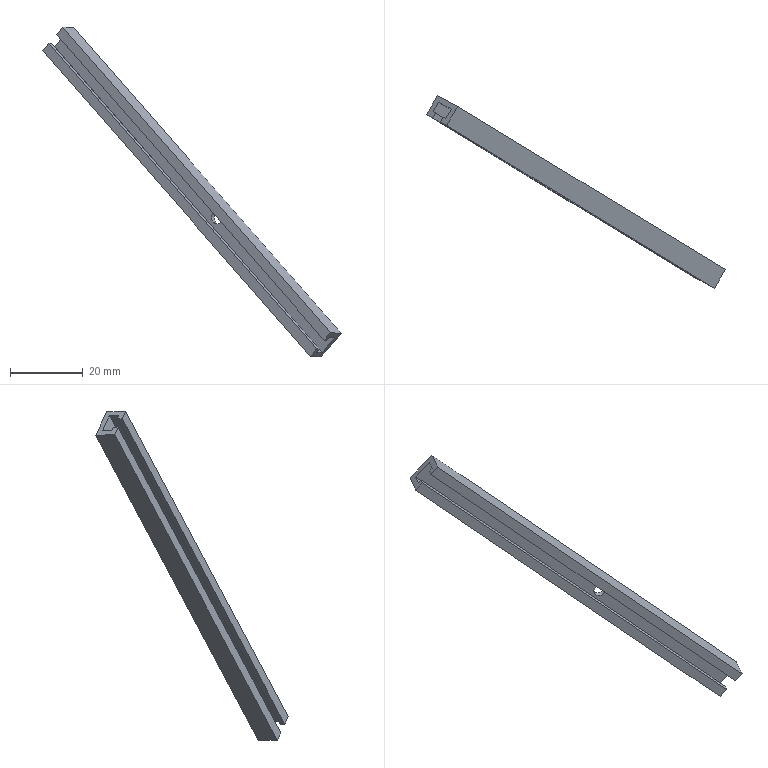Component | SolidWorks | KKSwitch-0710z0-123-1_SENA34H-400-V50-W150-X250-Y350-N3.5-0710z0-123-1 | 1 solid | 16 faces | box 81.95 x 52.78 x 90.38 mm | volume 3802 mm3 | plane 14 | cylinder 2 | commonest cylinder face diameters 3.5 x2
build123d program:
from build123d import *

# Parameters (mm, degrees)
BOSS_EXTRUDE1_DEPTH = 120
SKETCH2_R           = 1.75
CUT_EXTRUDE1_DEPTH  = 121.421


with BuildPart() as part:
    # Sketch1 → Boss-Extrude1 (new body)
    with BuildSketch(Plane.XY):
        Polygon((0, 0), (0, -2.8), (1.5, -2.8), (1.5, -1.65), (4.5, -1.65), (4.5, -7.35), (1.5, -7.35), (1.5, -6.2), (0, -6.2), (0, -9), (6, -9), (6, 0), align=None)
    extrude(amount=BOSS_EXTRUDE1_DEPTH)

    # Sketch2 → Cut-Extrude1 (cut, through all)
    with BuildSketch(Plane.ZY.offset(-4.5)):
        with Locations(Location((50, -4.5, 0), (0, 0, 270))):
            Circle(SKETCH2_R)
    extrude(amount=-CUT_EXTRUDE1_DEPTH, mode=Mode.SUBTRACT)


solid = part.part

# Placed as in the assembly
solid = solid.moved(Location((132.435, -51.049, 158.599), (-28.021, -37.728, 51.003)))
STEP:
#1=CARTESIAN_POINT('',(4.194,-1.11,7.69));
#2=VERTEX_POINT('',#1);
#3=CARTESIAN_POINT('',(4.278,-1.155,7.789));
#4=VERTEX_POINT('',#3);
#5=CARTESIAN_POINT('',(4.236,-1.132,7.739));
#6=DIRECTION('',(-0.4977,-0.867,0.02519));
#7=DIRECTION('',(0.6147,-0.3321,0.7154));
#8=AXIS2_PLACEMENT_3D('',#5,#6,#7);
#9=CIRCLE('',#8,0.0689);
#10=EDGE_CURVE('',#2,#4,#9,.T.);
#11=ORIENTED_EDGE('',*,*,#10,.F.);
#12=CARTESIAN_POINT('',(4.164,-1.161,7.691));
#13=VERTEX_POINT('',#12);
#14=CARTESIAN_POINT('',(4.194,-1.11,7.69));
#15=DIRECTION('',(-0.4977,-0.867,0.02519));
#16=VECTOR('',#15,39.37);
#17=LINE('',#14,#16);
#18=EDGE_CURVE('',#2,#13,#17,.T.);
#19=ORIENTED_EDGE('',*,*,#18,.T.);
#20=CARTESIAN_POINT('',(4.249,-1.206,7.79));
#21=VERTEX_POINT('',#20);
#22=CARTESIAN_POINT('',(4.207,-1.184,7.741));
#23=DIRECTION('',(-0.4977,-0.867,0.02519));
#24=DIRECTION('',(0.6147,-0.3321,0.7154));
#25=AXIS2_PLACEMENT_3D('',#22,#23,#24);
#26=CIRCLE('',#25,0.0689);
#27=EDGE_CURVE('',#13,#21,#26,.T.);
#28=ORIENTED_EDGE('',*,*,#27,.T.);
#29=CARTESIAN_POINT('',(4.278,-1.155,7.789));
#30=DIRECTION('',(-0.4977,-0.867,0.02519));
#31=VECTOR('',#30,39.37);
#32=LINE('',#29,#31);
#33=EDGE_CURVE('',#4,#21,#32,.T.);
#34=ORIENTED_EDGE('',*,*,#33,.F.);
#35=EDGE_LOOP('',(#11,#19,#28,#34));
#36=FACE_OUTER_BOUND('',#35,.T.);
#37=CARTESIAN_POINT('',(4.236,-1.132,7.739));
#38=DIRECTION('',(-0.4977,-0.867,0.02519));
#39=DIRECTION('',(0.6147,-0.3321,0.7154));
#40=AXIS2_PLACEMENT_3D('',#37,#38,#39);
#41=CYLINDRICAL_SURFACE('',#40,0.0689);
#42=ADVANCED_FACE('',(#36),#41,.F.);
#43=CARTESIAN_POINT('',(5.332,-1.805,6.238));
#44=VERTEX_POINT('',#43);
#45=CARTESIAN_POINT('',(5.214,-2.01,6.244));
#46=VERTEX_POINT('',#45);
#47=CARTESIAN_POINT('',(5.332,-1.805,6.238));
#48=DIRECTION('',(-0.4977,-0.867,0.02519));
#49=VECTOR('',#48,39.37);
#50=LINE('',#47,#49);
#51=EDGE_CURVE('',#44,#46,#50,.T.);
#52=ORIENTED_EDGE('',*,*,#51,.T.);
#53=CARTESIAN_POINT('',(2.323,-0.2543,9.543));
#54=VERTEX_POINT('',#53);
#55=CARTESIAN_POINT('',(2.323,-0.2543,9.543));
#56=DIRECTION('',(0.6119,-0.3716,-0.6982));
#57=VECTOR('',#56,39.37);
#58=LINE('',#55,#57);
#59=EDGE_CURVE('',#54,#46,#58,.T.);
#60=ORIENTED_EDGE('',*,*,#59,.F.);
#61=CARTESIAN_POINT('',(2.441,-0.04953,9.537));
#62=VERTEX_POINT('',#61);
#63=CARTESIAN_POINT('',(2.441,-0.04953,9.537));
#64=DIRECTION('',(-0.4977,-0.867,0.02519));
#65=VECTOR('',#64,39.37);
#66=LINE('',#63,#65);
#67=EDGE_CURVE('',#62,#54,#66,.T.);
#68=ORIENTED_EDGE('',*,*,#67,.F.);
#69=CARTESIAN_POINT('',(2.441,-0.04953,9.537));
#70=DIRECTION('',(0.6119,-0.3716,-0.6982));
#71=VECTOR('',#70,39.37);
#72=LINE('',#69,#71);
#73=EDGE_CURVE('',#62,#44,#72,.T.);
#74=ORIENTED_EDGE('',*,*,#73,.T.);
#75=EDGE_LOOP('',(#52,#60,#68,#74));
#76=FACE_OUTER_BOUND('',#75,.T.);
#77=CARTESIAN_POINT('',(2.441,-0.04953,9.537));
#78=DIRECTION('',(0.6147,-0.3321,0.7154));
#79=DIRECTION('',(0.6119,-0.3716,-0.6982));
#80=AXIS2_PLACEMENT_3D('',#77,#78,#79);
#81=PLANE('',#80);
#82=ADVANCED_FACE('',(#76),#81,.F.);
#83=CARTESIAN_POINT('',(5.282,-2.046,6.323));
#84=VERTEX_POINT('',#83);
#85=CARTESIAN_POINT('',(5.214,-2.01,6.244));
#86=DIRECTION('',(0.6147,-0.3321,0.7154));
#87=VECTOR('',#86,39.37);
#88=LINE('',#85,#87);
#89=EDGE_CURVE('',#46,#84,#88,.T.);
#90=ORIENTED_EDGE('',*,*,#89,.T.);
#91=CARTESIAN_POINT('',(2.391,-0.2909,9.622));
#92=VERTEX_POINT('',#91);
#93=CARTESIAN_POINT('',(2.391,-0.2909,9.622));
#94=DIRECTION('',(0.6119,-0.3716,-0.6982));
#95=VECTOR('',#94,39.37);
#96=LINE('',#93,#95);
#97=EDGE_CURVE('',#92,#84,#96,.T.);
#98=ORIENTED_EDGE('',*,*,#97,.F.);
#99=CARTESIAN_POINT('',(2.323,-0.2543,9.543));
#100=DIRECTION('',(0.6147,-0.3321,0.7154));
#101=VECTOR('',#100,39.37);
#102=LINE('',#99,#101);
#103=EDGE_CURVE('',#54,#92,#102,.T.);
#104=ORIENTED_EDGE('',*,*,#103,.F.);
#105=ORIENTED_EDGE('',*,*,#59,.T.);
#106=EDGE_LOOP('',(#90,#98,#104,#105));
#107=FACE_OUTER_BOUND('',#106,.T.);
#108=CARTESIAN_POINT('',(2.323,-0.2543,9.543));
#109=DIRECTION('',(0.4977,0.867,-0.02519));
#110=DIRECTION('',(0.6119,-0.3716,-0.6982));
#111=AXIS2_PLACEMENT_3D('',#108,#109,#110);
#112=PLANE('',#111);
#113=ADVANCED_FACE('',(#107),#112,.F.);
#114=CARTESIAN_POINT('',(5.311,-1.995,6.321));
#115=VERTEX_POINT('',#114);
#116=CARTESIAN_POINT('',(5.282,-2.046,6.323));
#117=DIRECTION('',(0.4977,0.867,-0.02519));
#118=VECTOR('',#117,39.37);
#119=LINE('',#116,#118);
#120=EDGE_CURVE('',#84,#115,#119,.T.);
#121=ORIENTED_EDGE('',*,*,#120,.T.);
#122=CARTESIAN_POINT('',(2.42,-0.2397,9.62));
#123=VERTEX_POINT('',#122);
#124=CARTESIAN_POINT('',(2.42,-0.2397,9.62));
#125=DIRECTION('',(0.6119,-0.3716,-0.6982));
#126=VECTOR('',#125,39.37);
#127=LINE('',#124,#126);
#128=EDGE_CURVE('',#123,#115,#127,.T.);
#129=ORIENTED_EDGE('',*,*,#128,.F.);
#130=CARTESIAN_POINT('',(2.391,-0.2909,9.622));
#131=DIRECTION('',(0.4977,0.867,-0.02519));
#132=VECTOR('',#131,39.37);
#133=LINE('',#130,#132);
#134=EDGE_CURVE('',#92,#123,#133,.T.);
#135=ORIENTED_EDGE('',*,*,#134,.F.);
#136=ORIENTED_EDGE('',*,*,#97,.T.);
#137=EDGE_LOOP('',(#121,#129,#135,#136));
#138=FACE_OUTER_BOUND('',#137,.T.);
#139=CARTESIAN_POINT('',(2.391,-0.2909,9.622));
#140=DIRECTION('',(-0.6147,0.3321,-0.7154));
#141=DIRECTION('',(-0.6119,0.3716,0.6982));
#142=AXIS2_PLACEMENT_3D('',#139,#140,#141);
#143=PLANE('',#142);
#144=ADVANCED_FACE('',(#138),#143,.F.);
#145=CARTESIAN_POINT('',(5.283,-1.98,6.289));
#146=VERTEX_POINT('',#145);
#147=CARTESIAN_POINT('',(5.311,-1.995,6.321));
#148=DIRECTION('',(-0.6147,0.3321,-0.7154));
#149=VECTOR('',#148,39.37);
#150=LINE('',#147,#149);
#151=EDGE_CURVE('',#115,#146,#150,.T.);
#152=ORIENTED_EDGE('',*,*,#151,.T.);
#153=CARTESIAN_POINT('',(2.392,-0.2247,9.588));
#154=VERTEX_POINT('',#153);
#155=CARTESIAN_POINT('',(2.392,-0.2247,9.588));
#156=DIRECTION('',(0.6119,-0.3716,-0.6982));
#157=VECTOR('',#156,39.37);
#158=LINE('',#155,#157);
#159=EDGE_CURVE('',#154,#146,#158,.T.);
#160=ORIENTED_EDGE('',*,*,#159,.F.);
#161=CARTESIAN_POINT('',(2.42,-0.2397,9.62));
#162=DIRECTION('',(-0.6147,0.3321,-0.7154));
#163=VECTOR('',#162,39.37);
#164=LINE('',#161,#163);
#165=EDGE_CURVE('',#123,#154,#164,.T.);
#166=ORIENTED_EDGE('',*,*,#165,.F.);
#167=ORIENTED_EDGE('',*,*,#128,.T.);
#168=EDGE_LOOP('',(#152,#160,#166,#167));
#169=FACE_OUTER_BOUND('',#168,.T.);
#170=CARTESIAN_POINT('',(2.42,-0.2397,9.62));
#171=DIRECTION('',(-0.4977,-0.867,0.02519));
#172=DIRECTION('',(-0.6119,0.3716,0.6982));
#173=AXIS2_PLACEMENT_3D('',#170,#171,#172);
#174=PLANE('',#173);
#175=ADVANCED_FACE('',(#169),#174,.F.);
#176=CARTESIAN_POINT('',(5.342,-1.878,6.286));
#177=VERTEX_POINT('',#176);
#178=CARTESIAN_POINT('',(5.283,-1.98,6.289));
#179=DIRECTION('',(0.4977,0.867,-0.02519));
#180=VECTOR('',#179,39.37);
#181=LINE('',#178,#180);
#182=EDGE_CURVE('',#146,#177,#181,.T.);
#183=ORIENTED_EDGE('',*,*,#182,.T.);
#184=CARTESIAN_POINT('',(2.451,-0.1223,9.585));
#185=VERTEX_POINT('',#184);
#186=CARTESIAN_POINT('',(2.451,-0.1223,9.585));
#187=DIRECTION('',(0.6119,-0.3716,-0.6982));
#188=VECTOR('',#187,39.37);
#189=LINE('',#186,#188);
#190=EDGE_CURVE('',#185,#177,#189,.T.);
#191=ORIENTED_EDGE('',*,*,#190,.F.);
#192=CARTESIAN_POINT('',(2.392,-0.2247,9.588));
#193=DIRECTION('',(0.4977,0.867,-0.02519));
#194=VECTOR('',#193,39.37);
#195=LINE('',#192,#194);
#196=EDGE_CURVE('',#154,#185,#195,.T.);
#197=ORIENTED_EDGE('',*,*,#196,.F.);
#198=ORIENTED_EDGE('',*,*,#159,.T.);
#199=EDGE_LOOP('',(#183,#191,#197,#198));
#200=FACE_OUTER_BOUND('',#199,.T.);
#201=CARTESIAN_POINT('',(2.392,-0.2247,9.588));
#202=DIRECTION('',(-0.6147,0.3321,-0.7154));
#203=DIRECTION('',(-0.6119,0.3716,0.6982));
#204=AXIS2_PLACEMENT_3D('',#201,#202,#203);
#205=PLANE('',#204);
#206=ADVANCED_FACE('',(#200),#205,.F.);
#207=CARTESIAN_POINT('',(4.207,-1.184,7.741));
#208=DIRECTION('',(-0.4977,-0.867,0.02519));
#209=DIRECTION('',(0.6147,-0.3321,0.7154));
#210=AXIS2_PLACEMENT_3D('',#207,#208,#209);
#211=CIRCLE('',#210,0.0689);
#212=EDGE_CURVE('',#21,#13,#211,.T.);
#213=ORIENTED_EDGE('',*,*,#212,.F.);
#214=ORIENTED_EDGE('',*,*,#27,.F.);
#215=EDGE_LOOP('',(#213,#214));
#216=FACE_BOUND('',#215,.T.);
#217=CARTESIAN_POINT('',(5.48,-1.952,6.447));
#218=VERTEX_POINT('',#217);
#219=CARTESIAN_POINT('',(5.342,-1.878,6.286));
#220=DIRECTION('',(0.6147,-0.3321,0.7154));
#221=VECTOR('',#220,39.37);
#222=LINE('',#219,#221);
#223=EDGE_CURVE('',#177,#218,#222,.T.);
#224=ORIENTED_EDGE('',*,*,#223,.T.);
#225=CARTESIAN_POINT('',(2.589,-0.1968,9.745));
#226=VERTEX_POINT('',#225);
#227=CARTESIAN_POINT('',(2.589,-0.1968,9.745));
#228=DIRECTION('',(0.6119,-0.3716,-0.6982));
#229=VECTOR('',#228,39.37);
#230=LINE('',#227,#229);
#231=EDGE_CURVE('',#226,#218,#230,.T.);
#232=ORIENTED_EDGE('',*,*,#231,.F.);
#233=CARTESIAN_POINT('',(2.451,-0.1223,9.585));
#234=DIRECTION('',(0.6147,-0.3321,0.7154));
#235=VECTOR('',#234,39.37);
#236=LINE('',#233,#235);
#237=EDGE_CURVE('',#185,#226,#236,.T.);
#238=ORIENTED_EDGE('',*,*,#237,.F.);
#239=ORIENTED_EDGE('',*,*,#190,.T.);
#240=EDGE_LOOP('',(#224,#232,#238,#239));
#241=FACE_OUTER_BOUND('',#240,.T.);
#242=CARTESIAN_POINT('',(2.451,-0.1223,9.585));
#243=DIRECTION('',(0.4977,0.867,-0.02519));
#244=DIRECTION('',(-0.6147,0.3321,-0.7154));
#245=AXIS2_PLACEMENT_3D('',#242,#243,#244);
#246=PLANE('',#245);
#247=ADVANCED_FACE('',(#216,#241),#246,.F.);
#248=CARTESIAN_POINT('',(5.421,-2.055,6.45));
#249=VERTEX_POINT('',#248);
#250=CARTESIAN_POINT('',(5.48,-1.952,6.447));
#251=DIRECTION('',(-0.4977,-0.867,0.02519));
#252=VECTOR('',#251,39.37);
#253=LINE('',#250,#252);
#254=EDGE_CURVE('',#218,#249,#253,.T.);
#255=ORIENTED_EDGE('',*,*,#254,.T.);
#256=CARTESIAN_POINT('',(2.53,-0.2992,9.748));
#257=VERTEX_POINT('',#256);
#258=CARTESIAN_POINT('',(2.53,-0.2992,9.748));
#259=DIRECTION('',(0.6119,-0.3716,-0.6982));
#260=VECTOR('',#259,39.37);
#261=LINE('',#258,#260);
#262=EDGE_CURVE('',#257,#249,#261,.T.);
#263=ORIENTED_EDGE('',*,*,#262,.F.);
#264=CARTESIAN_POINT('',(2.589,-0.1968,9.745));
#265=DIRECTION('',(-0.4977,-0.867,0.02519));
#266=VECTOR('',#265,39.37);
#267=LINE('',#264,#266);
#268=EDGE_CURVE('',#226,#257,#267,.T.);
#269=ORIENTED_EDGE('',*,*,#268,.F.);
#270=ORIENTED_EDGE('',*,*,#231,.T.);
#271=EDGE_LOOP('',(#255,#263,#269,#270));
#272=FACE_OUTER_BOUND('',#271,.T.);
#273=CARTESIAN_POINT('',(2.589,-0.1968,9.745));
#274=DIRECTION('',(0.6147,-0.3321,0.7154));
#275=DIRECTION('',(0.6119,-0.3716,-0.6982));
#276=AXIS2_PLACEMENT_3D('',#273,#274,#275);
#277=PLANE('',#276);
#278=ADVANCED_FACE('',(#272),#277,.F.);
#279=CARTESIAN_POINT('',(5.393,-2.04,6.417));
#280=VERTEX_POINT('',#279);
#281=CARTESIAN_POINT('',(5.421,-2.055,6.45));
#282=DIRECTION('',(-0.6147,0.3321,-0.7154));
#283=VECTOR('',#282,39.37);
#284=LINE('',#281,#283);
#285=EDGE_CURVE('',#249,#280,#284,.T.);
#286=ORIENTED_EDGE('',*,*,#285,.T.);
#287=CARTESIAN_POINT('',(2.503,-0.2842,9.716));
#288=VERTEX_POINT('',#287);
#289=CARTESIAN_POINT('',(2.503,-0.2842,9.716));
#290=DIRECTION('',(0.6119,-0.3716,-0.6982));
#291=VECTOR('',#290,39.37);
#292=LINE('',#289,#291);
#293=EDGE_CURVE('',#288,#280,#292,.T.);
#294=ORIENTED_EDGE('',*,*,#293,.F.);
#295=CARTESIAN_POINT('',(2.53,-0.2992,9.748));
#296=DIRECTION('',(-0.6147,0.3321,-0.7154));
#297=VECTOR('',#296,39.37);
#298=LINE('',#295,#297);
#299=EDGE_CURVE('',#257,#288,#298,.T.);
#300=ORIENTED_EDGE('',*,*,#299,.F.);
#301=ORIENTED_EDGE('',*,*,#262,.T.);
#302=EDGE_LOOP('',(#286,#294,#300,#301));
#303=FACE_OUTER_BOUND('',#302,.T.);
#304=CARTESIAN_POINT('',(2.53,-0.2992,9.748));
#305=DIRECTION('',(-0.4977,-0.867,0.02519));
#306=DIRECTION('',(-0.6119,0.3716,0.6982));
#307=AXIS2_PLACEMENT_3D('',#304,#305,#306);
#308=PLANE('',#307);
#309=ADVANCED_FACE('',(#303),#308,.F.);
#310=CARTESIAN_POINT('',(5.364,-2.091,6.419));
#311=VERTEX_POINT('',#310);
#312=CARTESIAN_POINT('',(5.393,-2.04,6.417));
#313=DIRECTION('',(-0.4977,-0.867,0.02519));
#314=VECTOR('',#313,39.37);
#315=LINE('',#312,#314);
#316=EDGE_CURVE('',#280,#311,#315,.T.);
#317=ORIENTED_EDGE('',*,*,#316,.T.);
#318=CARTESIAN_POINT('',(2.473,-0.3354,9.717));
#319=VERTEX_POINT('',#318);
#320=CARTESIAN_POINT('',(2.473,-0.3354,9.717));
#321=DIRECTION('',(0.6119,-0.3716,-0.6982));
#322=VECTOR('',#321,39.37);
#323=LINE('',#320,#322);
#324=EDGE_CURVE('',#319,#311,#323,.T.);
#325=ORIENTED_EDGE('',*,*,#324,.F.);
#326=CARTESIAN_POINT('',(2.503,-0.2842,9.716));
#327=DIRECTION('',(-0.4977,-0.867,0.02519));
#328=VECTOR('',#327,39.37);
#329=LINE('',#326,#328);
#330=EDGE_CURVE('',#288,#319,#329,.T.);
#331=ORIENTED_EDGE('',*,*,#330,.F.);
#332=ORIENTED_EDGE('',*,*,#293,.T.);
#333=EDGE_LOOP('',(#317,#325,#331,#332));
#334=FACE_OUTER_BOUND('',#333,.T.);
#335=CARTESIAN_POINT('',(2.503,-0.2842,9.716));
#336=DIRECTION('',(0.6147,-0.3321,0.7154));
#337=DIRECTION('',(0.6119,-0.3716,-0.6982));
#338=AXIS2_PLACEMENT_3D('',#335,#336,#337);
#339=PLANE('',#338);
#340=ADVANCED_FACE('',(#334),#339,.F.);
#341=CARTESIAN_POINT('',(5.432,-2.127,6.498));
#342=VERTEX_POINT('',#341);
#343=CARTESIAN_POINT('',(5.364,-2.091,6.419));
#344=DIRECTION('',(0.6147,-0.3321,0.7154));
#345=VECTOR('',#344,39.37);
#346=LINE('',#343,#345);
#347=EDGE_CURVE('',#311,#342,#346,.T.);
#348=ORIENTED_EDGE('',*,*,#347,.T.);
#349=CARTESIAN_POINT('',(2.541,-0.372,9.796));
#350=VERTEX_POINT('',#349);
#351=CARTESIAN_POINT('',(2.541,-0.372,9.796));
#352=DIRECTION('',(0.6119,-0.3716,-0.6982));
#353=VECTOR('',#352,39.37);
#354=LINE('',#351,#353);
#355=EDGE_CURVE('',#350,#342,#354,.T.);
#356=ORIENTED_EDGE('',*,*,#355,.F.);
#357=CARTESIAN_POINT('',(2.473,-0.3354,9.717));
#358=DIRECTION('',(0.6147,-0.3321,0.7154));
#359=VECTOR('',#358,39.37);
#360=LINE('',#357,#359);
#361=EDGE_CURVE('',#319,#350,#360,.T.);
#362=ORIENTED_EDGE('',*,*,#361,.F.);
#363=ORIENTED_EDGE('',*,*,#324,.T.);
#364=EDGE_LOOP('',(#348,#356,#362,#363));
#365=FACE_OUTER_BOUND('',#364,.T.);
#366=CARTESIAN_POINT('',(2.473,-0.3354,9.717));
#367=DIRECTION('',(0.4977,0.867,-0.02519));
#368=DIRECTION('',(0.6119,-0.3716,-0.6982));
#369=AXIS2_PLACEMENT_3D('',#366,#367,#368);
#370=PLANE('',#369);
#371=ADVANCED_FACE('',(#365),#370,.F.);
#372=CARTESIAN_POINT('',(5.549,-1.923,6.492));
#373=VERTEX_POINT('',#372);
#374=CARTESIAN_POINT('',(5.432,-2.127,6.498));
#375=DIRECTION('',(0.4977,0.867,-0.02519));
#376=VECTOR('',#375,39.37);
#377=LINE('',#374,#376);
#378=EDGE_CURVE('',#342,#373,#377,.T.);
#379=ORIENTED_EDGE('',*,*,#378,.T.);
#380=CARTESIAN_POINT('',(2.658,-0.1672,9.79));
#381=VERTEX_POINT('',#380);
#382=CARTESIAN_POINT('',(2.658,-0.1672,9.79));
#383=DIRECTION('',(0.6119,-0.3716,-0.6982));
#384=VECTOR('',#383,39.37);
#385=LINE('',#382,#384);
#386=EDGE_CURVE('',#381,#373,#385,.T.);
#387=ORIENTED_EDGE('',*,*,#386,.F.);
#388=CARTESIAN_POINT('',(2.541,-0.372,9.796));
#389=DIRECTION('',(0.4977,0.867,-0.02519));
#390=VECTOR('',#389,39.37);
#391=LINE('',#388,#390);
#392=EDGE_CURVE('',#350,#381,#391,.T.);
#393=ORIENTED_EDGE('',*,*,#392,.F.);
#394=ORIENTED_EDGE('',*,*,#355,.T.);
#395=EDGE_LOOP('',(#379,#387,#393,#394));
#396=FACE_OUTER_BOUND('',#395,.T.);
#397=CARTESIAN_POINT('',(2.541,-0.372,9.796));
#398=DIRECTION('',(-0.6147,0.3321,-0.7154));
#399=DIRECTION('',(-0.6119,0.3716,0.6982));
#400=AXIS2_PLACEMENT_3D('',#397,#398,#399);
#401=PLANE('',#400);
#402=ADVANCED_FACE('',(#396),#401,.F.);
#403=CARTESIAN_POINT('',(4.236,-1.132,7.739));
#404=DIRECTION('',(-0.4977,-0.867,0.02519));
#405=DIRECTION('',(0.6147,-0.3321,0.7154));
#406=AXIS2_PLACEMENT_3D('',#403,#404,#405);
#407=CIRCLE('',#406,0.0689);
#408=EDGE_CURVE('',#4,#2,#407,.T.);
#409=ORIENTED_EDGE('',*,*,#408,.T.);
#410=ORIENTED_EDGE('',*,*,#10,.T.);
#411=EDGE_LOOP('',(#409,#410));
#412=FACE_BOUND('',#411,.T.);
#413=CARTESIAN_POINT('',(5.549,-1.923,6.492));
#414=DIRECTION('',(-0.6147,0.3321,-0.7154));
#415=VECTOR('',#414,39.37);
#416=LINE('',#413,#415);
#417=EDGE_CURVE('',#373,#44,#416,.T.);
#418=ORIENTED_EDGE('',*,*,#417,.T.);
#419=ORIENTED_EDGE('',*,*,#73,.F.);
#420=CARTESIAN_POINT('',(2.658,-0.1672,9.79));
#421=DIRECTION('',(-0.6147,0.3321,-0.7154));
#422=VECTOR('',#421,39.37);
#423=LINE('',#420,#422);
#424=EDGE_CURVE('',#381,#62,#423,.T.);
#425=ORIENTED_EDGE('',*,*,#424,.F.);
#426=ORIENTED_EDGE('',*,*,#386,.T.);
#427=EDGE_LOOP('',(#418,#419,#425,#426));
#428=FACE_OUTER_BOUND('',#427,.T.);
#429=CARTESIAN_POINT('',(2.658,-0.1672,9.79));
#430=DIRECTION('',(-0.4977,-0.867,0.02519));
#431=DIRECTION('',(-0.6119,0.3716,0.6982));
#432=AXIS2_PLACEMENT_3D('',#429,#430,#431);
#433=PLANE('',#432);
#434=ADVANCED_FACE('',(#412,#428),#433,.F.);
#435=ORIENTED_EDGE('',*,*,#67,.T.);
#436=ORIENTED_EDGE('',*,*,#103,.T.);
#437=ORIENTED_EDGE('',*,*,#134,.T.);
#438=ORIENTED_EDGE('',*,*,#165,.T.);
#439=ORIENTED_EDGE('',*,*,#196,.T.);
#440=ORIENTED_EDGE('',*,*,#237,.T.);
#441=ORIENTED_EDGE('',*,*,#268,.T.);
#442=ORIENTED_EDGE('',*,*,#299,.T.);
#443=ORIENTED_EDGE('',*,*,#330,.T.);
#444=ORIENTED_EDGE('',*,*,#361,.T.);
#445=ORIENTED_EDGE('',*,*,#392,.T.);
#446=ORIENTED_EDGE('',*,*,#424,.T.);
#447=EDGE_LOOP('',(#435,#436,#437,#438,#439,#440,#441,#442,#443,#444,#445,#446));
#448=FACE_OUTER_BOUND('',#447,.T.);
#449=CARTESIAN_POINT('',(2.323,-0.2543,9.543));
#450=DIRECTION('',(-0.6119,0.3716,0.6982));
#451=DIRECTION('',(0.4977,0.867,-0.02519));
#452=AXIS2_PLACEMENT_3D('',#449,#450,#451);
#453=PLANE('',#452);
#454=ADVANCED_FACE('',(#448),#453,.T.);
#455=ORIENTED_EDGE('',*,*,#51,.F.);
#456=ORIENTED_EDGE('',*,*,#417,.F.);
#457=ORIENTED_EDGE('',*,*,#378,.F.);
#458=ORIENTED_EDGE('',*,*,#347,.F.);
#459=ORIENTED_EDGE('',*,*,#316,.F.);
#460=ORIENTED_EDGE('',*,*,#285,.F.);
#461=ORIENTED_EDGE('',*,*,#254,.F.);
#462=ORIENTED_EDGE('',*,*,#223,.F.);
#463=ORIENTED_EDGE('',*,*,#182,.F.);
#464=ORIENTED_EDGE('',*,*,#151,.F.);
#465=ORIENTED_EDGE('',*,*,#120,.F.);
#466=ORIENTED_EDGE('',*,*,#89,.F.);
#467=EDGE_LOOP('',(#455,#456,#457,#458,#459,#460,#461,#462,#463,#464,#465,#466));
#468=FACE_OUTER_BOUND('',#467,.T.);
#469=CARTESIAN_POINT('',(5.214,-2.01,6.244));
#470=DIRECTION('',(-0.6119,0.3716,0.6982));
#471=DIRECTION('',(0.4977,0.867,-0.02519));
#472=AXIS2_PLACEMENT_3D('',#469,#470,#471);
#473=PLANE('',#472);
#474=ADVANCED_FACE('',(#468),#473,.F.);
#475=ORIENTED_EDGE('',*,*,#18,.F.);
#476=ORIENTED_EDGE('',*,*,#408,.F.);
#477=ORIENTED_EDGE('',*,*,#33,.T.);
#478=ORIENTED_EDGE('',*,*,#212,.T.);
#479=EDGE_LOOP('',(#475,#476,#477,#478));
#480=FACE_OUTER_BOUND('',#479,.T.);
#481=CARTESIAN_POINT('',(4.236,-1.132,7.739));
#482=DIRECTION('',(-0.4977,-0.867,0.02519));
#483=DIRECTION('',(0.6147,-0.3321,0.7154));
#484=AXIS2_PLACEMENT_3D('',#481,#482,#483);
#485=CYLINDRICAL_SURFACE('',#484,0.0689);
#486=ADVANCED_FACE('',(#480),#485,.F.);
#487=CLOSED_SHELL('',(#42,#82,#113,#144,#175,#206,#247,#278,#309,#340,#371,#402,#434,#454,#474,#486));
#488=MANIFOLD_SOLID_BREP('',#487);
#489=CARTESIAN_POINT('',(0.,0.,0.));
#490=DIRECTION('',(0.,0.,1.));
#491=DIRECTION('',(1.,0.,0.));
#492=AXIS2_PLACEMENT_3D('',#489,#490,#491);
#493=(LENGTH_UNIT()NAMED_UNIT(*)SI_UNIT($,.METRE.));
#494=LENGTH_MEASURE_WITH_UNIT(LENGTH_MEASURE(0.0254),#493);
#495=DIMENSIONAL_EXPONENTS(1.,0.,0.,0.,0.,0.,0.);
#496=(CONVERSION_BASED_UNIT('',#494)LENGTH_UNIT()NAMED_UNIT(#495));
#497=UNCERTAINTY_MEASURE_WITH_UNIT(LENGTH_MEASURE(0.00001),#496,'','');
#498=(NAMED_UNIT(*)PLANE_ANGLE_UNIT()SI_UNIT($,.RADIAN.));
#499=(NAMED_UNIT(*)SI_UNIT($,.STERADIAN.)SOLID_ANGLE_UNIT());
#500=(GEOMETRIC_REPRESENTATION_CONTEXT(3)GLOBAL_UNCERTAINTY_ASSIGNED_CONTEXT((#497))GLOBAL_UNIT_ASSIGNED_CONTEXT((#496,#498,#499))REPRESENTATION_CONTEXT('',''));
#501=ADVANCED_BREP_SHAPE_REPRESENTATION('',(#488,#492),#500);
#502=COLOUR_RGB('',0.7922,0.8196,0.9333);
#503=FILL_AREA_STYLE_COLOUR('',#502);
#504=FILL_AREA_STYLE('',(#503));
#505=SURFACE_STYLE_FILL_AREA(#504);
#506=SURFACE_SIDE_STYLE('',(#505));
#507=SURFACE_STYLE_USAGE(.BOTH.,#506);
#508=PRESENTATION_STYLE_ASSIGNMENT((#507));
#509=STYLED_ITEM('',(#508),#488);
#510=PRESENTATION_LAYER_ASSIGNMENT('','',(#509));
#511=(LENGTH_UNIT()NAMED_UNIT(*)SI_UNIT($,.METRE.));
#512=LENGTH_MEASURE_WITH_UNIT(LENGTH_MEASURE(0.0254),#511);
#513=DIMENSIONAL_EXPONENTS(1.,0.,0.,0.,0.,0.,0.);
#514=(CONVERSION_BASED_UNIT('',#512)LENGTH_UNIT()NAMED_UNIT(#513));
#515=UNCERTAINTY_MEASURE_WITH_UNIT(LENGTH_MEASURE(0.00001),#514,'','');
#516=(NAMED_UNIT(*)PLANE_ANGLE_UNIT()SI_UNIT($,.RADIAN.));
#517=(NAMED_UNIT(*)SI_UNIT($,.STERADIAN.)SOLID_ANGLE_UNIT());
#518=(GEOMETRIC_REPRESENTATION_CONTEXT(3)GLOBAL_UNCERTAINTY_ASSIGNED_CONTEXT((#515))GLOBAL_UNIT_ASSIGNED_CONTEXT((#514,#516,#517))REPRESENTATION_CONTEXT('',''));
#519=MECHANICAL_DESIGN_GEOMETRIC_PRESENTATION_REPRESENTATION('',(#509),#518);